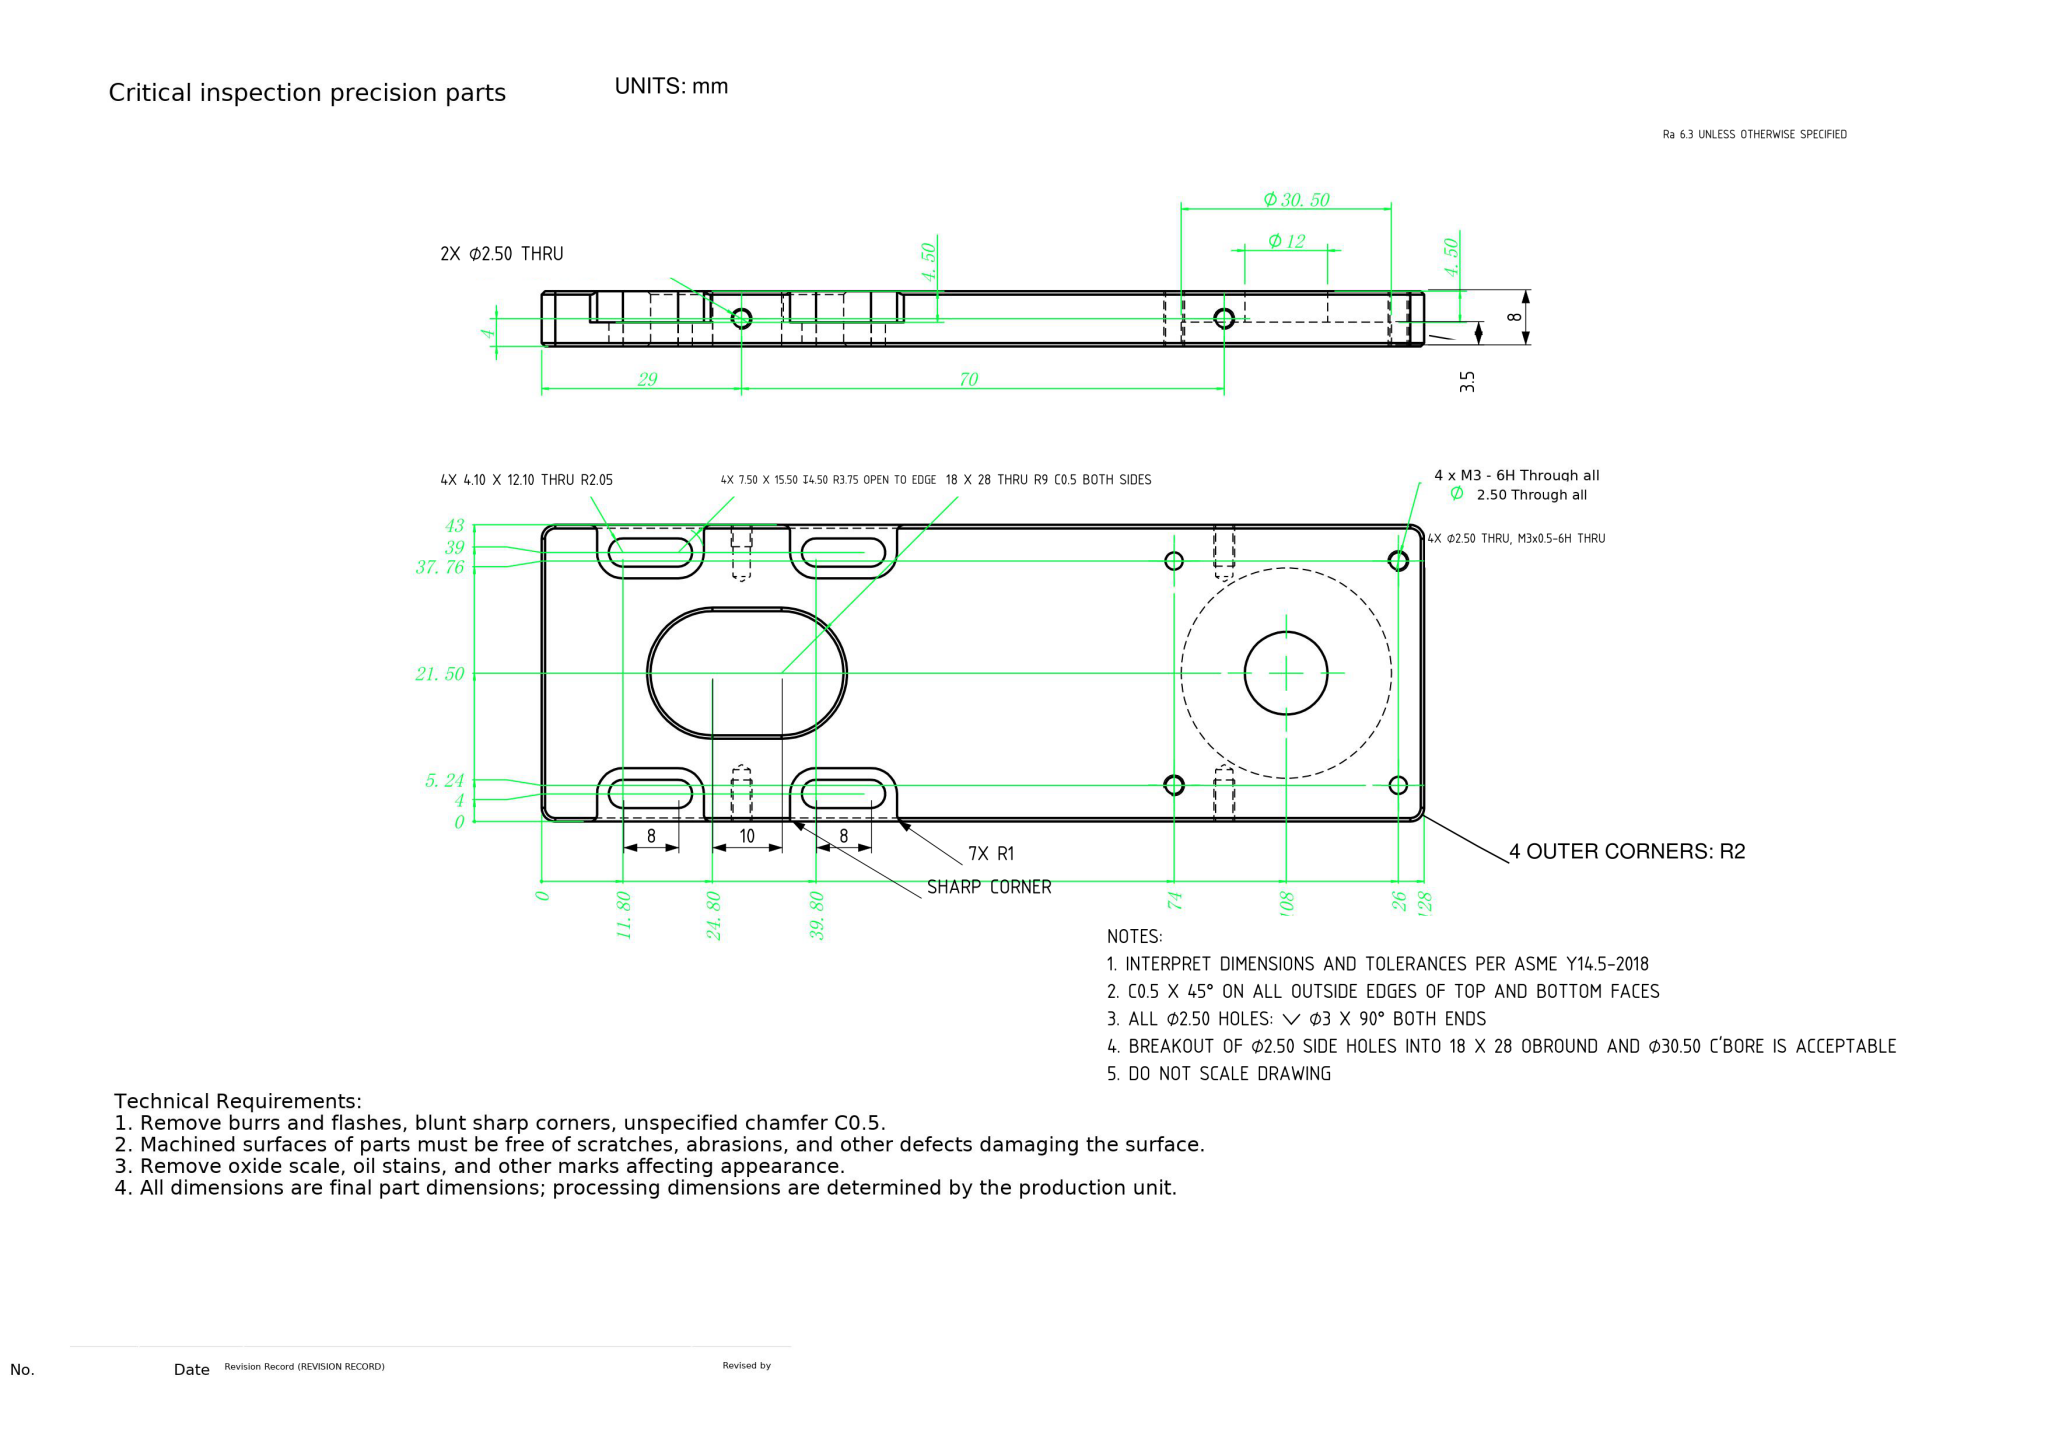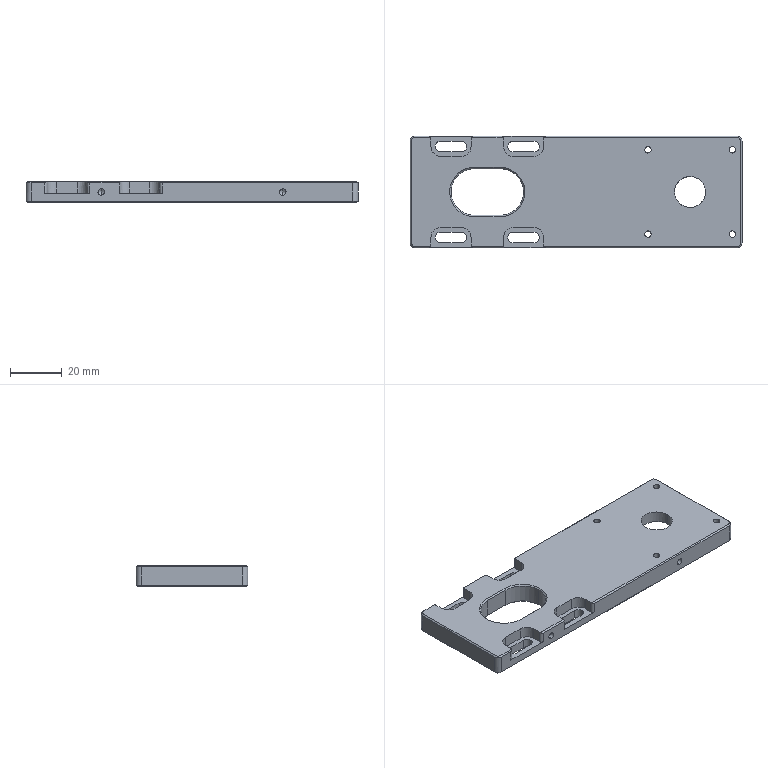Part | NX | mm | 1 solid | 125 faces | box 128 x 43 x 8 mm | volume 34354 mm3 | cylinder 54 | plane 49 | cone 22 | commonest cylinder face diameters 2.5 x16 4.1 x12 7.5 x8 2 x7 4 x4 18 x3 30.5 x2 12 x2